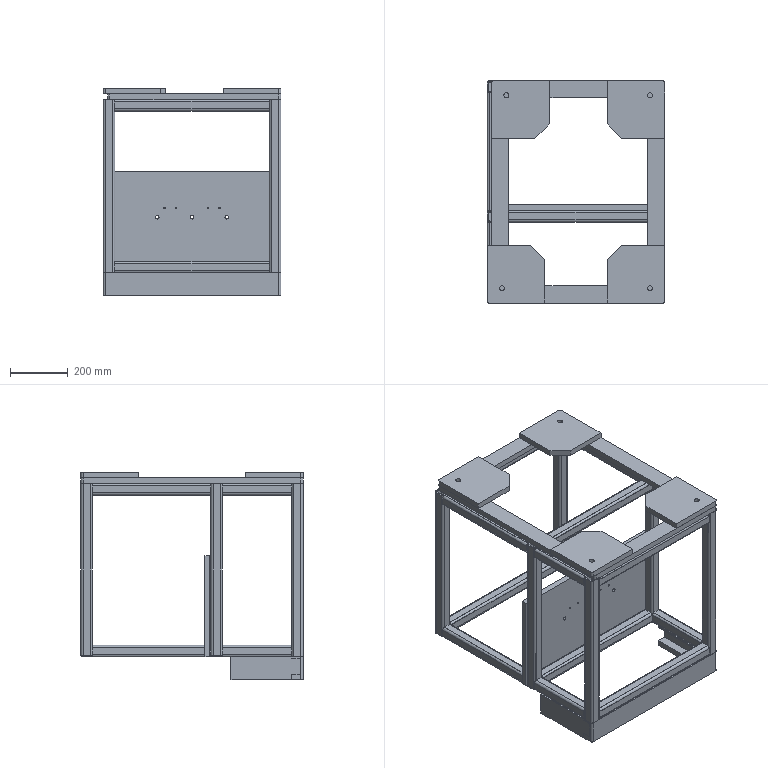Component | SolidWorks | STRack-1 | 33 solids | 527 faces | volume 17028559 mm3 | plane 322 | cylinder 205 | commonest cylinder face diameters 16 x90 8 x80 12 x12 17.5 x8 5 x8 20 x4 6 x3